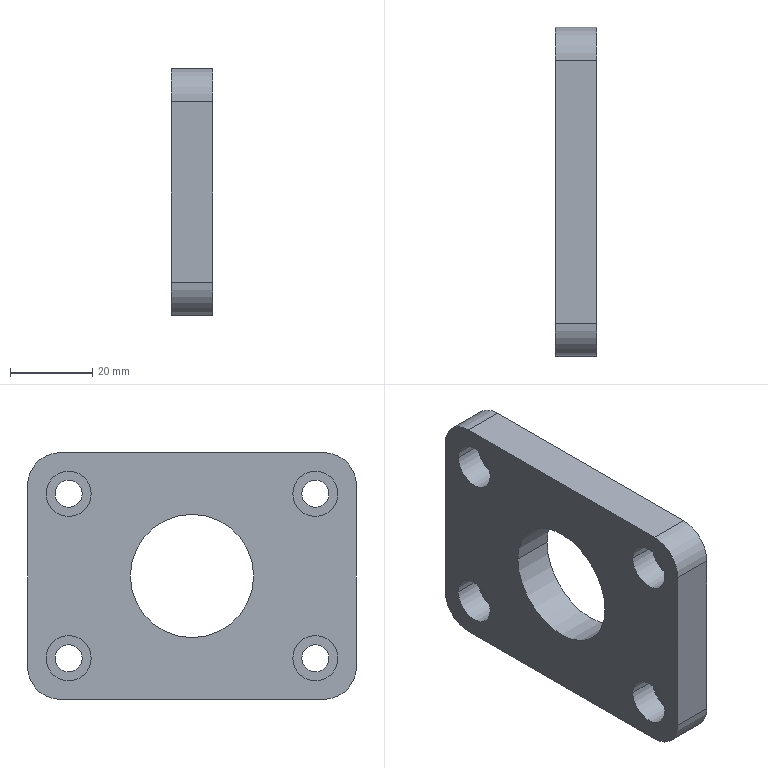Component | SolidWorks | GuideWheelAssembly-2_GuideWheelBracket-1_GuideWheelBracketPlate-1 | 1 solid | 32 faces | box 10 x 80 x 60 mm | volume 37359 mm3 | cylinder 22 | plane 10 | commonest cylinder face diameters 11 x8 6.6 x8 16 x4 30 x2 | material Nylon 101
build123d program:
from build123d import *

# Parameters (mm, degrees)
SKETCH1_W                                            = 80
SKETCH1_H                                            = 60
BOSS_EXTRUDE1_DEPTH                                  = 10
FILLET1_R                                            = 8
HOLE_SIZE_ACCORDING_TO_THE_TYPE_OF_HEXAG_D           = 6.6
HOLE_SIZE_ACCORDING_TO_THE_TYPE_OF_HEXAG_CBORE_D     = 11
HOLE_SIZE_ACCORDING_TO_THE_TYPE_OF_HEXAG_CBORE_DEPTH = 6.8
SKETCH4_R                                            = 15
CUT_EXTRUDE1_DEPTH                                   = 10


with BuildPart() as part:
    # Sketch1 → Boss-Extrude1 (new body)
    with BuildSketch(Plane.XY):
        Rectangle(SKETCH1_W, SKETCH1_H)
    extrude(amount=BOSS_EXTRUDE1_DEPTH)

    # Fillet1
    fillet1_edges = [part.edges().sort_by_distance(p)[0] for p in [
        (40, -30, 5),
        (-40, -30, 5),
        (-40, 30, 5),
        (40, 30, 5),
    ]]
    fillet(fillet1_edges, radius=FILLET1_R)

    # Hole Size according to the type of Hexag (through all)
    with Locations(Plane.XY.offset(10)):
        with Locations((-30, 20), (30, 20), (-30, -20), (30, -20)):
            CounterBoreHole(HOLE_SIZE_ACCORDING_TO_THE_TYPE_OF_HEXAG_D / 2, HOLE_SIZE_ACCORDING_TO_THE_TYPE_OF_HEXAG_CBORE_D / 2, HOLE_SIZE_ACCORDING_TO_THE_TYPE_OF_HEXAG_CBORE_DEPTH)

    # Sketch4 → Cut-Extrude1 (cut)
    with BuildSketch(Plane.XY.offset(10)):
        Circle(SKETCH4_R)
    extrude(amount=-CUT_EXTRUDE1_DEPTH, mode=Mode.SUBTRACT)


solid = part.part

# Placed as in the assembly
solid = solid.moved(Location((-510, 0, 305), (90, -90, 0)))
STEP:
#1=COLOUR_RGB('',0.7922,0.8196,0.9333);
#2=FILL_AREA_STYLE_COLOUR('',#1);
#3=FILL_AREA_STYLE('',(#2));
#4=SURFACE_STYLE_FILL_AREA(#3);
#5=SURFACE_SIDE_STYLE('',(#4));
#6=SURFACE_STYLE_USAGE(.BOTH.,#5);
#7=PRESENTATION_STYLE_ASSIGNMENT((#6));
#8=CARTESIAN_POINT('',(-20.079,0.5906,12.008));
#9=VERTEX_POINT('',#8);
#10=CARTESIAN_POINT('',(-20.079,-0.5906,12.008));
#11=VERTEX_POINT('',#10);
#12=CARTESIAN_POINT('',(-20.079,-0.,12.008));
#13=DIRECTION('',(-1.,0.,-0.));
#14=DIRECTION('',(0.,-1.,0.));
#15=AXIS2_PLACEMENT_3D('',#12,#13,#14);
#16=CIRCLE('',#15,0.5906);
#17=EDGE_CURVE('',#9,#11,#16,.T.);
#18=ORIENTED_EDGE('',*,*,#17,.F.);
#19=CARTESIAN_POINT('',(-20.472,0.5906,12.008));
#20=VERTEX_POINT('',#19);
#21=CARTESIAN_POINT('',(-20.079,0.5906,12.008));
#22=DIRECTION('',(-1.,0.,-0.));
#23=VECTOR('',#22,39.37);
#24=LINE('',#21,#23);
#25=EDGE_CURVE('',#9,#20,#24,.T.);
#26=ORIENTED_EDGE('',*,*,#25,.T.);
#27=CARTESIAN_POINT('',(-20.472,-0.5906,12.008));
#28=VERTEX_POINT('',#27);
#29=CARTESIAN_POINT('',(-20.472,-0.,12.008));
#30=DIRECTION('',(-1.,0.,-0.));
#31=DIRECTION('',(0.,-1.,0.));
#32=AXIS2_PLACEMENT_3D('',#29,#30,#31);
#33=CIRCLE('',#32,0.5906);
#34=EDGE_CURVE('',#20,#28,#33,.T.);
#35=ORIENTED_EDGE('',*,*,#34,.T.);
#36=CARTESIAN_POINT('',(-20.079,-0.5906,12.008));
#37=DIRECTION('',(-1.,0.,-0.));
#38=VECTOR('',#37,39.37);
#39=LINE('',#36,#38);
#40=EDGE_CURVE('',#11,#28,#39,.T.);
#41=ORIENTED_EDGE('',*,*,#40,.F.);
#42=EDGE_LOOP('',(#18,#26,#35,#41));
#43=FACE_OUTER_BOUND('',#42,.T.);
#44=CARTESIAN_POINT('',(-20.079,-0.,12.008));
#45=DIRECTION('',(-1.,0.,-0.));
#46=DIRECTION('',(0.,-1.,0.));
#47=AXIS2_PLACEMENT_3D('',#44,#45,#46);
#48=CYLINDRICAL_SURFACE('',#47,0.5906);
#49=ADVANCED_FACE('',(#43),#48,.F.);
#50=CARTESIAN_POINT('',(-20.205,1.398,12.795));
#51=VERTEX_POINT('',#50);
#52=CARTESIAN_POINT('',(-20.205,0.9646,12.795));
#53=VERTEX_POINT('',#52);
#54=CARTESIAN_POINT('',(-20.205,1.181,12.795));
#55=DIRECTION('',(-1.,0.,-0.));
#56=DIRECTION('',(0.,-1.,0.));
#57=AXIS2_PLACEMENT_3D('',#54,#55,#56);
#58=CIRCLE('',#57,0.2165);
#59=EDGE_CURVE('',#51,#53,#58,.T.);
#60=ORIENTED_EDGE('',*,*,#59,.F.);
#61=CARTESIAN_POINT('',(-20.472,1.398,12.795));
#62=VERTEX_POINT('',#61);
#63=CARTESIAN_POINT('',(-20.472,1.398,12.795));
#64=DIRECTION('',(-1.,0.,-0.));
#65=VECTOR('',#64,39.37);
#66=LINE('',#63,#65);
#67=EDGE_CURVE('',#51,#62,#66,.T.);
#68=ORIENTED_EDGE('',*,*,#67,.T.);
#69=CARTESIAN_POINT('',(-20.472,0.9646,12.795));
#70=VERTEX_POINT('',#69);
#71=CARTESIAN_POINT('',(-20.472,1.181,12.795));
#72=DIRECTION('',(-1.,0.,-0.));
#73=DIRECTION('',(0.,-1.,0.));
#74=AXIS2_PLACEMENT_3D('',#71,#72,#73);
#75=CIRCLE('',#74,0.2165);
#76=EDGE_CURVE('',#62,#70,#75,.T.);
#77=ORIENTED_EDGE('',*,*,#76,.T.);
#78=CARTESIAN_POINT('',(-20.472,0.9646,12.795));
#79=DIRECTION('',(-1.,0.,-0.));
#80=VECTOR('',#79,39.37);
#81=LINE('',#78,#80);
#82=EDGE_CURVE('',#53,#70,#81,.T.);
#83=ORIENTED_EDGE('',*,*,#82,.F.);
#84=EDGE_LOOP('',(#60,#68,#77,#83));
#85=FACE_OUTER_BOUND('',#84,.T.);
#86=CARTESIAN_POINT('',(-20.472,1.181,12.795));
#87=DIRECTION('',(-1.,0.,-0.));
#88=DIRECTION('',(0.,-1.,0.));
#89=AXIS2_PLACEMENT_3D('',#86,#87,#88);
#90=CYLINDRICAL_SURFACE('',#89,0.2165);
#91=ADVANCED_FACE('',(#85),#90,.F.);
#92=CARTESIAN_POINT('',(-20.079,1.311,12.795));
#93=VERTEX_POINT('',#92);
#94=CARTESIAN_POINT('',(-20.079,1.051,12.795));
#95=VERTEX_POINT('',#94);
#96=CARTESIAN_POINT('',(-20.079,1.181,12.795));
#97=DIRECTION('',(-1.,0.,-0.));
#98=DIRECTION('',(0.,-1.,0.));
#99=AXIS2_PLACEMENT_3D('',#96,#97,#98);
#100=CIRCLE('',#99,0.1299);
#101=EDGE_CURVE('',#93,#95,#100,.T.);
#102=ORIENTED_EDGE('',*,*,#101,.F.);
#103=CARTESIAN_POINT('',(-20.205,1.311,12.795));
#104=VERTEX_POINT('',#103);
#105=CARTESIAN_POINT('',(-20.472,1.311,12.795));
#106=DIRECTION('',(-1.,0.,-0.));
#107=VECTOR('',#106,39.37);
#108=LINE('',#105,#107);
#109=EDGE_CURVE('',#93,#104,#108,.T.);
#110=ORIENTED_EDGE('',*,*,#109,.T.);
#111=CARTESIAN_POINT('',(-20.205,1.051,12.795));
#112=VERTEX_POINT('',#111);
#113=CARTESIAN_POINT('',(-20.205,1.181,12.795));
#114=DIRECTION('',(-1.,0.,-0.));
#115=DIRECTION('',(0.,-1.,0.));
#116=AXIS2_PLACEMENT_3D('',#113,#114,#115);
#117=CIRCLE('',#116,0.1299);
#118=EDGE_CURVE('',#104,#112,#117,.T.);
#119=ORIENTED_EDGE('',*,*,#118,.T.);
#120=CARTESIAN_POINT('',(-20.472,1.051,12.795));
#121=DIRECTION('',(-1.,0.,-0.));
#122=VECTOR('',#121,39.37);
#123=LINE('',#120,#122);
#124=EDGE_CURVE('',#95,#112,#123,.T.);
#125=ORIENTED_EDGE('',*,*,#124,.F.);
#126=EDGE_LOOP('',(#102,#110,#119,#125));
#127=FACE_OUTER_BOUND('',#126,.T.);
#128=CARTESIAN_POINT('',(-20.472,1.181,12.795));
#129=DIRECTION('',(-1.,0.,-0.));
#130=DIRECTION('',(0.,-1.,0.));
#131=AXIS2_PLACEMENT_3D('',#128,#129,#130);
#132=CYLINDRICAL_SURFACE('',#131,0.1299);
#133=ADVANCED_FACE('',(#127),#132,.F.);
#134=CARTESIAN_POINT('',(-20.205,-0.9646,12.795));
#135=VERTEX_POINT('',#134);
#136=CARTESIAN_POINT('',(-20.205,-1.398,12.795));
#137=VERTEX_POINT('',#136);
#138=CARTESIAN_POINT('',(-20.205,-1.181,12.795));
#139=DIRECTION('',(-1.,0.,-0.));
#140=DIRECTION('',(0.,-1.,0.));
#141=AXIS2_PLACEMENT_3D('',#138,#139,#140);
#142=CIRCLE('',#141,0.2165);
#143=EDGE_CURVE('',#135,#137,#142,.T.);
#144=ORIENTED_EDGE('',*,*,#143,.F.);
#145=CARTESIAN_POINT('',(-20.472,-0.9646,12.795));
#146=VERTEX_POINT('',#145);
#147=CARTESIAN_POINT('',(-20.472,-0.9646,12.795));
#148=DIRECTION('',(-1.,0.,-0.));
#149=VECTOR('',#148,39.37);
#150=LINE('',#147,#149);
#151=EDGE_CURVE('',#135,#146,#150,.T.);
#152=ORIENTED_EDGE('',*,*,#151,.T.);
#153=CARTESIAN_POINT('',(-20.472,-1.398,12.795));
#154=VERTEX_POINT('',#153);
#155=CARTESIAN_POINT('',(-20.472,-1.181,12.795));
#156=DIRECTION('',(-1.,0.,-0.));
#157=DIRECTION('',(0.,-1.,0.));
#158=AXIS2_PLACEMENT_3D('',#155,#156,#157);
#159=CIRCLE('',#158,0.2165);
#160=EDGE_CURVE('',#146,#154,#159,.T.);
#161=ORIENTED_EDGE('',*,*,#160,.T.);
#162=CARTESIAN_POINT('',(-20.472,-1.398,12.795));
#163=DIRECTION('',(-1.,0.,-0.));
#164=VECTOR('',#163,39.37);
#165=LINE('',#162,#164);
#166=EDGE_CURVE('',#137,#154,#165,.T.);
#167=ORIENTED_EDGE('',*,*,#166,.F.);
#168=EDGE_LOOP('',(#144,#152,#161,#167));
#169=FACE_OUTER_BOUND('',#168,.T.);
#170=CARTESIAN_POINT('',(-20.472,-1.181,12.795));
#171=DIRECTION('',(-1.,0.,-0.));
#172=DIRECTION('',(0.,-1.,0.));
#173=AXIS2_PLACEMENT_3D('',#170,#171,#172);
#174=CYLINDRICAL_SURFACE('',#173,0.2165);
#175=ADVANCED_FACE('',(#169),#174,.F.);
#176=CARTESIAN_POINT('',(-20.079,-1.051,12.795));
#177=VERTEX_POINT('',#176);
#178=CARTESIAN_POINT('',(-20.079,-1.311,12.795));
#179=VERTEX_POINT('',#178);
#180=CARTESIAN_POINT('',(-20.079,-1.181,12.795));
#181=DIRECTION('',(-1.,0.,-0.));
#182=DIRECTION('',(0.,-1.,0.));
#183=AXIS2_PLACEMENT_3D('',#180,#181,#182);
#184=CIRCLE('',#183,0.1299);
#185=EDGE_CURVE('',#177,#179,#184,.T.);
#186=ORIENTED_EDGE('',*,*,#185,.F.);
#187=CARTESIAN_POINT('',(-20.205,-1.051,12.795));
#188=VERTEX_POINT('',#187);
#189=CARTESIAN_POINT('',(-20.472,-1.051,12.795));
#190=DIRECTION('',(-1.,0.,-0.));
#191=VECTOR('',#190,39.37);
#192=LINE('',#189,#191);
#193=EDGE_CURVE('',#177,#188,#192,.T.);
#194=ORIENTED_EDGE('',*,*,#193,.T.);
#195=CARTESIAN_POINT('',(-20.205,-1.311,12.795));
#196=VERTEX_POINT('',#195);
#197=CARTESIAN_POINT('',(-20.205,-1.181,12.795));
#198=DIRECTION('',(-1.,0.,-0.));
#199=DIRECTION('',(0.,-1.,0.));
#200=AXIS2_PLACEMENT_3D('',#197,#198,#199);
#201=CIRCLE('',#200,0.1299);
#202=EDGE_CURVE('',#188,#196,#201,.T.);
#203=ORIENTED_EDGE('',*,*,#202,.T.);
#204=CARTESIAN_POINT('',(-20.472,-1.311,12.795));
#205=DIRECTION('',(-1.,0.,-0.));
#206=VECTOR('',#205,39.37);
#207=LINE('',#204,#206);
#208=EDGE_CURVE('',#179,#196,#207,.T.);
#209=ORIENTED_EDGE('',*,*,#208,.F.);
#210=EDGE_LOOP('',(#186,#194,#203,#209));
#211=FACE_OUTER_BOUND('',#210,.T.);
#212=CARTESIAN_POINT('',(-20.472,-1.181,12.795));
#213=DIRECTION('',(-1.,0.,-0.));
#214=DIRECTION('',(0.,-1.,0.));
#215=AXIS2_PLACEMENT_3D('',#212,#213,#214);
#216=CYLINDRICAL_SURFACE('',#215,0.1299);
#217=ADVANCED_FACE('',(#211),#216,.F.);
#218=CARTESIAN_POINT('',(-20.205,1.398,11.22));
#219=VERTEX_POINT('',#218);
#220=CARTESIAN_POINT('',(-20.205,0.9646,11.22));
#221=VERTEX_POINT('',#220);
#222=CARTESIAN_POINT('',(-20.205,1.181,11.22));
#223=DIRECTION('',(-1.,0.,-0.));
#224=DIRECTION('',(0.,-1.,0.));
#225=AXIS2_PLACEMENT_3D('',#222,#223,#224);
#226=CIRCLE('',#225,0.2165);
#227=EDGE_CURVE('',#219,#221,#226,.T.);
#228=ORIENTED_EDGE('',*,*,#227,.F.);
#229=CARTESIAN_POINT('',(-20.472,1.398,11.22));
#230=VERTEX_POINT('',#229);
#231=CARTESIAN_POINT('',(-20.472,1.398,11.22));
#232=DIRECTION('',(-1.,0.,-0.));
#233=VECTOR('',#232,39.37);
#234=LINE('',#231,#233);
#235=EDGE_CURVE('',#219,#230,#234,.T.);
#236=ORIENTED_EDGE('',*,*,#235,.T.);
#237=CARTESIAN_POINT('',(-20.472,0.9646,11.22));
#238=VERTEX_POINT('',#237);
#239=CARTESIAN_POINT('',(-20.472,1.181,11.22));
#240=DIRECTION('',(-1.,0.,-0.));
#241=DIRECTION('',(0.,-1.,0.));
#242=AXIS2_PLACEMENT_3D('',#239,#240,#241);
#243=CIRCLE('',#242,0.2165);
#244=EDGE_CURVE('',#230,#238,#243,.T.);
#245=ORIENTED_EDGE('',*,*,#244,.T.);
#246=CARTESIAN_POINT('',(-20.472,0.9646,11.22));
#247=DIRECTION('',(-1.,0.,-0.));
#248=VECTOR('',#247,39.37);
#249=LINE('',#246,#248);
#250=EDGE_CURVE('',#221,#238,#249,.T.);
#251=ORIENTED_EDGE('',*,*,#250,.F.);
#252=EDGE_LOOP('',(#228,#236,#245,#251));
#253=FACE_OUTER_BOUND('',#252,.T.);
#254=CARTESIAN_POINT('',(-20.472,1.181,11.22));
#255=DIRECTION('',(-1.,0.,-0.));
#256=DIRECTION('',(0.,-1.,0.));
#257=AXIS2_PLACEMENT_3D('',#254,#255,#256);
#258=CYLINDRICAL_SURFACE('',#257,0.2165);
#259=ADVANCED_FACE('',(#253),#258,.F.);
#260=CARTESIAN_POINT('',(-20.079,1.311,11.22));
#261=VERTEX_POINT('',#260);
#262=CARTESIAN_POINT('',(-20.079,1.051,11.22));
#263=VERTEX_POINT('',#262);
#264=CARTESIAN_POINT('',(-20.079,1.181,11.22));
#265=DIRECTION('',(-1.,0.,-0.));
#266=DIRECTION('',(0.,-1.,0.));
#267=AXIS2_PLACEMENT_3D('',#264,#265,#266);
#268=CIRCLE('',#267,0.1299);
#269=EDGE_CURVE('',#261,#263,#268,.T.);
#270=ORIENTED_EDGE('',*,*,#269,.F.);
#271=CARTESIAN_POINT('',(-20.205,1.311,11.22));
#272=VERTEX_POINT('',#271);
#273=CARTESIAN_POINT('',(-20.472,1.311,11.22));
#274=DIRECTION('',(-1.,0.,-0.));
#275=VECTOR('',#274,39.37);
#276=LINE('',#273,#275);
#277=EDGE_CURVE('',#261,#272,#276,.T.);
#278=ORIENTED_EDGE('',*,*,#277,.T.);
#279=CARTESIAN_POINT('',(-20.205,1.051,11.22));
#280=VERTEX_POINT('',#279);
#281=CARTESIAN_POINT('',(-20.205,1.181,11.22));
#282=DIRECTION('',(-1.,0.,-0.));
#283=DIRECTION('',(0.,-1.,0.));
#284=AXIS2_PLACEMENT_3D('',#281,#282,#283);
#285=CIRCLE('',#284,0.1299);
#286=EDGE_CURVE('',#272,#280,#285,.T.);
#287=ORIENTED_EDGE('',*,*,#286,.T.);
#288=CARTESIAN_POINT('',(-20.472,1.051,11.22));
#289=DIRECTION('',(-1.,0.,-0.));
#290=VECTOR('',#289,39.37);
#291=LINE('',#288,#290);
#292=EDGE_CURVE('',#263,#280,#291,.T.);
#293=ORIENTED_EDGE('',*,*,#292,.F.);
#294=EDGE_LOOP('',(#270,#278,#287,#293));
#295=FACE_OUTER_BOUND('',#294,.T.);
#296=CARTESIAN_POINT('',(-20.472,1.181,11.22));
#297=DIRECTION('',(-1.,0.,-0.));
#298=DIRECTION('',(0.,-1.,0.));
#299=AXIS2_PLACEMENT_3D('',#296,#297,#298);
#300=CYLINDRICAL_SURFACE('',#299,0.1299);
#301=ADVANCED_FACE('',(#295),#300,.F.);
#302=CARTESIAN_POINT('',(-20.205,-0.9646,11.22));
#303=VERTEX_POINT('',#302);
#304=CARTESIAN_POINT('',(-20.205,-1.398,11.22));
#305=VERTEX_POINT('',#304);
#306=CARTESIAN_POINT('',(-20.205,-1.181,11.22));
#307=DIRECTION('',(-1.,0.,-0.));
#308=DIRECTION('',(0.,-1.,0.));
#309=AXIS2_PLACEMENT_3D('',#306,#307,#308);
#310=CIRCLE('',#309,0.2165);
#311=EDGE_CURVE('',#303,#305,#310,.T.);
#312=ORIENTED_EDGE('',*,*,#311,.F.);
#313=CARTESIAN_POINT('',(-20.472,-0.9646,11.22));
#314=VERTEX_POINT('',#313);
#315=CARTESIAN_POINT('',(-20.472,-0.9646,11.22));
#316=DIRECTION('',(-1.,0.,-0.));
#317=VECTOR('',#316,39.37);
#318=LINE('',#315,#317);
#319=EDGE_CURVE('',#303,#314,#318,.T.);
#320=ORIENTED_EDGE('',*,*,#319,.T.);
#321=CARTESIAN_POINT('',(-20.472,-1.398,11.22));
#322=VERTEX_POINT('',#321);
#323=CARTESIAN_POINT('',(-20.472,-1.181,11.22));
#324=DIRECTION('',(-1.,0.,-0.));
#325=DIRECTION('',(0.,-1.,0.));
#326=AXIS2_PLACEMENT_3D('',#323,#324,#325);
#327=CIRCLE('',#326,0.2165);
#328=EDGE_CURVE('',#314,#322,#327,.T.);
#329=ORIENTED_EDGE('',*,*,#328,.T.);
#330=CARTESIAN_POINT('',(-20.472,-1.398,11.22));
#331=DIRECTION('',(-1.,0.,-0.));
#332=VECTOR('',#331,39.37);
#333=LINE('',#330,#332);
#334=EDGE_CURVE('',#305,#322,#333,.T.);
#335=ORIENTED_EDGE('',*,*,#334,.F.);
#336=EDGE_LOOP('',(#312,#320,#329,#335));
#337=FACE_OUTER_BOUND('',#336,.T.);
#338=CARTESIAN_POINT('',(-20.472,-1.181,11.22));
#339=DIRECTION('',(-1.,0.,-0.));
#340=DIRECTION('',(0.,-1.,0.));
#341=AXIS2_PLACEMENT_3D('',#338,#339,#340);
#342=CYLINDRICAL_SURFACE('',#341,0.2165);
#343=ADVANCED_FACE('',(#337),#342,.F.);
#344=CARTESIAN_POINT('',(-20.079,-1.051,11.22));
#345=VERTEX_POINT('',#344);
#346=CARTESIAN_POINT('',(-20.079,-1.311,11.22));
#347=VERTEX_POINT('',#346);
#348=CARTESIAN_POINT('',(-20.079,-1.181,11.22));
#349=DIRECTION('',(-1.,0.,-0.));
#350=DIRECTION('',(0.,-1.,0.));
#351=AXIS2_PLACEMENT_3D('',#348,#349,#350);
#352=CIRCLE('',#351,0.1299);
#353=EDGE_CURVE('',#345,#347,#352,.T.);
#354=ORIENTED_EDGE('',*,*,#353,.F.);
#355=CARTESIAN_POINT('',(-20.205,-1.051,11.22));
#356=VERTEX_POINT('',#355);
#357=CARTESIAN_POINT('',(-20.472,-1.051,11.22));
#358=DIRECTION('',(-1.,0.,-0.));
#359=VECTOR('',#358,39.37);
#360=LINE('',#357,#359);
#361=EDGE_CURVE('',#345,#356,#360,.T.);
#362=ORIENTED_EDGE('',*,*,#361,.T.);
#363=CARTESIAN_POINT('',(-20.205,-1.311,11.22));
#364=VERTEX_POINT('',#363);
#365=CARTESIAN_POINT('',(-20.205,-1.181,11.22));
#366=DIRECTION('',(-1.,0.,-0.));
#367=DIRECTION('',(0.,-1.,0.));
#368=AXIS2_PLACEMENT_3D('',#365,#366,#367);
#369=CIRCLE('',#368,0.1299);
#370=EDGE_CURVE('',#356,#364,#369,.T.);
#371=ORIENTED_EDGE('',*,*,#370,.T.);
#372=CARTESIAN_POINT('',(-20.472,-1.311,11.22));
#373=DIRECTION('',(-1.,0.,-0.));
#374=VECTOR('',#373,39.37);
#375=LINE('',#372,#374);
#376=EDGE_CURVE('',#347,#364,#375,.T.);
#377=ORIENTED_EDGE('',*,*,#376,.F.);
#378=EDGE_LOOP('',(#354,#362,#371,#377));
#379=FACE_OUTER_BOUND('',#378,.T.);
#380=CARTESIAN_POINT('',(-20.472,-1.181,11.22));
#381=DIRECTION('',(-1.,0.,-0.));
#382=DIRECTION('',(0.,-1.,0.));
#383=AXIS2_PLACEMENT_3D('',#380,#381,#382);
#384=CYLINDRICAL_SURFACE('',#383,0.1299);
#385=ADVANCED_FACE('',(#379),#384,.F.);
#386=CARTESIAN_POINT('',(-20.472,-1.575,11.142));
#387=VERTEX_POINT('',#386);
#388=CARTESIAN_POINT('',(-20.472,-1.575,12.874));
#389=VERTEX_POINT('',#388);
#390=CARTESIAN_POINT('',(-20.472,-1.575,13.189));
#391=DIRECTION('',(-0.,-0.,1.));
#392=VECTOR('',#391,39.37);
#393=LINE('',#390,#392);
#394=EDGE_CURVE('',#387,#389,#393,.T.);
#395=ORIENTED_EDGE('',*,*,#394,.F.);
#396=CARTESIAN_POINT('',(-20.079,-1.575,11.142));
#397=VERTEX_POINT('',#396);
#398=CARTESIAN_POINT('',(-20.472,-1.575,11.142));
#399=DIRECTION('',(1.,-0.,0.));
#400=VECTOR('',#399,39.37);
#401=LINE('',#398,#400);
#402=EDGE_CURVE('',#387,#397,#401,.T.);
#403=ORIENTED_EDGE('',*,*,#402,.T.);
#404=CARTESIAN_POINT('',(-20.079,-1.575,12.874));
#405=VERTEX_POINT('',#404);
#406=CARTESIAN_POINT('',(-20.079,-1.575,13.189));
#407=DIRECTION('',(-0.,-0.,1.));
#408=VECTOR('',#407,39.37);
#409=LINE('',#406,#408);
#410=EDGE_CURVE('',#397,#405,#409,.T.);
#411=ORIENTED_EDGE('',*,*,#410,.T.);
#412=CARTESIAN_POINT('',(-20.472,-1.575,12.874));
#413=DIRECTION('',(-1.,0.,-0.));
#414=VECTOR('',#413,39.37);
#415=LINE('',#412,#414);
#416=EDGE_CURVE('',#405,#389,#415,.T.);
#417=ORIENTED_EDGE('',*,*,#416,.T.);
#418=EDGE_LOOP('',(#395,#403,#411,#417));
#419=FACE_OUTER_BOUND('',#418,.T.);
#420=CARTESIAN_POINT('',(-20.472,-1.575,13.189));
#421=DIRECTION('',(-0.,1.,0.));
#422=DIRECTION('',(0.,0.,-1.));
#423=AXIS2_PLACEMENT_3D('',#420,#421,#422);
#424=PLANE('',#423);
#425=ADVANCED_FACE('',(#419),#424,.F.);
#426=CARTESIAN_POINT('',(-20.079,-1.26,13.189));
#427=VERTEX_POINT('',#426);
#428=CARTESIAN_POINT('',(-20.079,1.26,13.189));
#429=VERTEX_POINT('',#428);
#430=CARTESIAN_POINT('',(-20.079,1.575,13.189));
#431=DIRECTION('',(-0.,1.,0.));
#432=VECTOR('',#431,39.37);
#433=LINE('',#430,#432);
#434=EDGE_CURVE('',#427,#429,#433,.T.);
#435=ORIENTED_EDGE('',*,*,#434,.T.);
#436=CARTESIAN_POINT('',(-20.472,1.26,13.189));
#437=VERTEX_POINT('',#436);
#438=CARTESIAN_POINT('',(-20.472,1.26,13.189));
#439=DIRECTION('',(-1.,0.,-0.));
#440=VECTOR('',#439,39.37);
#441=LINE('',#438,#440);
#442=EDGE_CURVE('',#429,#437,#441,.T.);
#443=ORIENTED_EDGE('',*,*,#442,.T.);
#444=CARTESIAN_POINT('',(-20.472,-1.26,13.189));
#445=VERTEX_POINT('',#444);
#446=CARTESIAN_POINT('',(-20.472,1.575,13.189));
#447=DIRECTION('',(-0.,1.,0.));
#448=VECTOR('',#447,39.37);
#449=LINE('',#446,#448);
#450=EDGE_CURVE('',#445,#437,#449,.T.);
#451=ORIENTED_EDGE('',*,*,#450,.F.);
#452=CARTESIAN_POINT('',(-20.472,-1.26,13.189));
#453=DIRECTION('',(1.,-0.,0.));
#454=VECTOR('',#453,39.37);
#455=LINE('',#452,#454);
#456=EDGE_CURVE('',#445,#427,#455,.T.);
#457=ORIENTED_EDGE('',*,*,#456,.T.);
#458=EDGE_LOOP('',(#435,#443,#451,#457));
#459=FACE_OUTER_BOUND('',#458,.T.);
#460=CARTESIAN_POINT('',(-20.472,1.575,13.189));
#461=DIRECTION('',(0.,0.,-1.));
#462=DIRECTION('',(1.,-0.,0.));
#463=AXIS2_PLACEMENT_3D('',#460,#461,#462);
#464=PLANE('',#463);
#465=ADVANCED_FACE('',(#459),#464,.F.);
#466=CARTESIAN_POINT('',(-20.079,1.575,12.874));
#467=VERTEX_POINT('',#466);
#468=CARTESIAN_POINT('',(-20.079,1.575,11.142));
#469=VERTEX_POINT('',#468);
#470=CARTESIAN_POINT('',(-20.079,1.575,13.189));
#471=DIRECTION('',(0.,0.,-1.));
#472=VECTOR('',#471,39.37);
#473=LINE('',#470,#472);
#474=EDGE_CURVE('',#467,#469,#473,.T.);
#475=ORIENTED_EDGE('',*,*,#474,.T.);
#476=CARTESIAN_POINT('',(-20.472,1.575,11.142));
#477=VERTEX_POINT('',#476);
#478=CARTESIAN_POINT('',(-20.472,1.575,11.142));
#479=DIRECTION('',(-1.,0.,-0.));
#480=VECTOR('',#479,39.37);
#481=LINE('',#478,#480);
#482=EDGE_CURVE('',#469,#477,#481,.T.);
#483=ORIENTED_EDGE('',*,*,#482,.T.);
#484=CARTESIAN_POINT('',(-20.472,1.575,12.874));
#485=VERTEX_POINT('',#484);
#486=CARTESIAN_POINT('',(-20.472,1.575,13.189));
#487=DIRECTION('',(0.,0.,-1.));
#488=VECTOR('',#487,39.37);
#489=LINE('',#486,#488);
#490=EDGE_CURVE('',#485,#477,#489,.T.);
#491=ORIENTED_EDGE('',*,*,#490,.F.);
#492=CARTESIAN_POINT('',(-20.472,1.575,12.874));
#493=DIRECTION('',(1.,-0.,0.));
#494=VECTOR('',#493,39.37);
#495=LINE('',#492,#494);
#496=EDGE_CURVE('',#485,#467,#495,.T.);
#497=ORIENTED_EDGE('',*,*,#496,.T.);
#498=EDGE_LOOP('',(#475,#483,#491,#497));
#499=FACE_OUTER_BOUND('',#498,.T.);
#500=CARTESIAN_POINT('',(-20.472,1.575,13.189));
#501=DIRECTION('',(0.,-1.,-0.));
#502=DIRECTION('',(-0.,-0.,1.));
#503=AXIS2_PLACEMENT_3D('',#500,#501,#502);
#504=PLANE('',#503);
#505=ADVANCED_FACE('',(#499),#504,.F.);
#506=CARTESIAN_POINT('',(-20.079,1.26,10.827));
#507=VERTEX_POINT('',#506);
#508=CARTESIAN_POINT('',(-20.079,-1.26,10.827));
#509=VERTEX_POINT('',#508);
#510=CARTESIAN_POINT('',(-20.079,1.575,10.827));
#511=DIRECTION('',(0.,-1.,-0.));
#512=VECTOR('',#511,39.37);
#513=LINE('',#510,#512);
#514=EDGE_CURVE('',#507,#509,#513,.T.);
#515=ORIENTED_EDGE('',*,*,#514,.T.);
#516=CARTESIAN_POINT('',(-20.472,-1.26,10.827));
#517=VERTEX_POINT('',#516);
#518=CARTESIAN_POINT('',(-20.472,-1.26,10.827));
#519=DIRECTION('',(-1.,0.,-0.));
#520=VECTOR('',#519,39.37);
#521=LINE('',#518,#520);
#522=EDGE_CURVE('',#509,#517,#521,.T.);
#523=ORIENTED_EDGE('',*,*,#522,.T.);
#524=CARTESIAN_POINT('',(-20.472,1.26,10.827));
#525=VERTEX_POINT('',#524);
#526=CARTESIAN_POINT('',(-20.472,1.575,10.827));
#527=DIRECTION('',(0.,-1.,-0.));
#528=VECTOR('',#527,39.37);
#529=LINE('',#526,#528);
#530=EDGE_CURVE('',#525,#517,#529,.T.);
#531=ORIENTED_EDGE('',*,*,#530,.F.);
#532=CARTESIAN_POINT('',(-20.472,1.26,10.827));
#533=DIRECTION('',(1.,-0.,0.));
#534=VECTOR('',#533,39.37);
#535=LINE('',#532,#534);
#536=EDGE_CURVE('',#525,#507,#535,.T.);
#537=ORIENTED_EDGE('',*,*,#536,.T.);
#538=EDGE_LOOP('',(#515,#523,#531,#537));
#539=FACE_OUTER_BOUND('',#538,.T.);
#540=CARTESIAN_POINT('',(-20.472,1.575,10.827));
#541=DIRECTION('',(-0.,-0.,1.));
#542=DIRECTION('',(-1.,0.,-0.));
#543=AXIS2_PLACEMENT_3D('',#540,#541,#542);
#544=PLANE('',#543);
#545=ADVANCED_FACE('',(#539),#544,.F.);
#546=CARTESIAN_POINT('',(-20.472,-0.,12.008));
#547=DIRECTION('',(-1.,0.,-0.));
#548=DIRECTION('',(0.,-1.,0.));
#549=AXIS2_PLACEMENT_3D('',#546,#547,#548);
#550=CIRCLE('',#549,0.5906);
#551=EDGE_CURVE('',#28,#20,#550,.T.);
#552=ORIENTED_EDGE('',*,*,#551,.F.);
#553=ORIENTED_EDGE('',*,*,#34,.F.);
#554=EDGE_LOOP('',(#552,#553));
#555=FACE_BOUND('',#554,.T.);
#556=CARTESIAN_POINT('',(-20.472,1.181,12.795));
#557=DIRECTION('',(-1.,0.,-0.));
#558=DIRECTION('',(0.,-1.,0.));
#559=AXIS2_PLACEMENT_3D('',#556,#557,#558);
#560=CIRCLE('',#559,0.2165);
#561=EDGE_CURVE('',#70,#62,#560,.T.);
#562=ORIENTED_EDGE('',*,*,#561,.F.);
#563=ORIENTED_EDGE('',*,*,#76,.F.);
#564=EDGE_LOOP('',(#562,#563));
#565=FACE_BOUND('',#564,.T.);
#566=CARTESIAN_POINT('',(-20.472,-1.181,12.795));
#567=DIRECTION('',(-1.,0.,-0.));
#568=DIRECTION('',(0.,-1.,0.));
#569=AXIS2_PLACEMENT_3D('',#566,#567,#568);
#570=CIRCLE('',#569,0.2165);
#571=EDGE_CURVE('',#154,#146,#570,.T.);
#572=ORIENTED_EDGE('',*,*,#571,.F.);
#573=ORIENTED_EDGE('',*,*,#160,.F.);
#574=EDGE_LOOP('',(#572,#573));
#575=FACE_BOUND('',#574,.T.);
#576=CARTESIAN_POINT('',(-20.472,1.181,11.22));
#577=DIRECTION('',(-1.,0.,-0.));
#578=DIRECTION('',(0.,-1.,0.));
#579=AXIS2_PLACEMENT_3D('',#576,#577,#578);
#580=CIRCLE('',#579,0.2165);
#581=EDGE_CURVE('',#238,#230,#580,.T.);
#582=ORIENTED_EDGE('',*,*,#581,.F.);
#583=ORIENTED_EDGE('',*,*,#244,.F.);
#584=EDGE_LOOP('',(#582,#583));
#585=FACE_BOUND('',#584,.T.);
#586=CARTESIAN_POINT('',(-20.472,-1.181,11.22));
#587=DIRECTION('',(-1.,0.,-0.));
#588=DIRECTION('',(0.,-1.,0.));
#589=AXIS2_PLACEMENT_3D('',#586,#587,#588);
#590=CIRCLE('',#589,0.2165);
#591=EDGE_CURVE('',#322,#314,#590,.T.);
#592=ORIENTED_EDGE('',*,*,#591,.F.);
#593=ORIENTED_EDGE('',*,*,#328,.F.);
#594=EDGE_LOOP('',(#592,#593));
#595=FACE_BOUND('',#594,.T.);
#596=ORIENTED_EDGE('',*,*,#530,.T.);
#597=CARTESIAN_POINT('',(-20.472,-1.26,11.142));
#598=DIRECTION('',(-1.,0.,-0.));
#599=DIRECTION('',(0.,-1.,0.));
#600=AXIS2_PLACEMENT_3D('',#597,#598,#599);
#601=CIRCLE('',#600,0.315);
#602=EDGE_CURVE('',#517,#387,#601,.T.);
#603=ORIENTED_EDGE('',*,*,#602,.T.);
#604=ORIENTED_EDGE('',*,*,#394,.T.);
#605=CARTESIAN_POINT('',(-20.472,-1.26,12.874));
#606=DIRECTION('',(-1.,0.,-0.));
#607=DIRECTION('',(0.,-1.,0.));
#608=AXIS2_PLACEMENT_3D('',#605,#606,#607);
#609=CIRCLE('',#608,0.315);
#610=EDGE_CURVE('',#389,#445,#609,.T.);
#611=ORIENTED_EDGE('',*,*,#610,.T.);
#612=ORIENTED_EDGE('',*,*,#450,.T.);
#613=CARTESIAN_POINT('',(-20.472,1.26,12.874));
#614=DIRECTION('',(-1.,0.,-0.));
#615=DIRECTION('',(0.,-1.,0.));
#616=AXIS2_PLACEMENT_3D('',#613,#614,#615);
#617=CIRCLE('',#616,0.315);
#618=EDGE_CURVE('',#437,#485,#617,.T.);
#619=ORIENTED_EDGE('',*,*,#618,.T.);
#620=ORIENTED_EDGE('',*,*,#490,.T.);
#621=CARTESIAN_POINT('',(-20.472,1.26,11.142));
#622=DIRECTION('',(-1.,0.,-0.));
#623=DIRECTION('',(0.,-1.,0.));
#624=AXIS2_PLACEMENT_3D('',#621,#622,#623);
#625=CIRCLE('',#624,0.315);
#626=EDGE_CURVE('',#477,#525,#625,.T.);
#627=ORIENTED_EDGE('',*,*,#626,.T.);
#628=EDGE_LOOP('',(#596,#603,#604,#611,#612,#619,#620,#627));
#629=FACE_OUTER_BOUND('',#628,.T.);
#630=CARTESIAN_POINT('',(-20.472,-0.,12.008));
#631=DIRECTION('',(-1.,-0.,-0.));
#632=DIRECTION('',(0.,-1.,-0.));
#633=AXIS2_PLACEMENT_3D('',#630,#631,#632);
#634=PLANE('',#633);
#635=ADVANCED_FACE('',(#555,#565,#575,#585,#595,#629),#634,.T.);
#636=CARTESIAN_POINT('',(-20.079,-0.,12.008));
#637=DIRECTION('',(-1.,0.,-0.));
#638=DIRECTION('',(0.,-1.,0.));
#639=AXIS2_PLACEMENT_3D('',#636,#637,#638);
#640=CIRCLE('',#639,0.5906);
#641=EDGE_CURVE('',#11,#9,#640,.T.);
#642=ORIENTED_EDGE('',*,*,#641,.T.);
#643=ORIENTED_EDGE('',*,*,#17,.T.);
#644=EDGE_LOOP('',(#642,#643));
#645=FACE_BOUND('',#644,.T.);
#646=CARTESIAN_POINT('',(-20.079,1.181,12.795));
#647=DIRECTION('',(-1.,0.,-0.));
#648=DIRECTION('',(0.,-1.,0.));
#649=AXIS2_PLACEMENT_3D('',#646,#647,#648);
#650=CIRCLE('',#649,0.1299);
#651=EDGE_CURVE('',#95,#93,#650,.T.);
#652=ORIENTED_EDGE('',*,*,#651,.T.);
#653=ORIENTED_EDGE('',*,*,#101,.T.);
#654=EDGE_LOOP('',(#652,#653));
#655=FACE_BOUND('',#654,.T.);
#656=CARTESIAN_POINT('',(-20.079,-1.181,12.795));
#657=DIRECTION('',(-1.,0.,-0.));
#658=DIRECTION('',(0.,-1.,0.));
#659=AXIS2_PLACEMENT_3D('',#656,#657,#658);
#660=CIRCLE('',#659,0.1299);
#661=EDGE_CURVE('',#179,#177,#660,.T.);
#662=ORIENTED_EDGE('',*,*,#661,.T.);
#663=ORIENTED_EDGE('',*,*,#185,.T.);
#664=EDGE_LOOP('',(#662,#663));
#665=FACE_BOUND('',#664,.T.);
#666=CARTESIAN_POINT('',(-20.079,1.181,11.22));
#667=DIRECTION('',(-1.,0.,-0.));
#668=DIRECTION('',(0.,-1.,0.));
#669=AXIS2_PLACEMENT_3D('',#666,#667,#668);
#670=CIRCLE('',#669,0.1299);
#671=EDGE_CURVE('',#263,#261,#670,.T.);
#672=ORIENTED_EDGE('',*,*,#671,.T.);
#673=ORIENTED_EDGE('',*,*,#269,.T.);
#674=EDGE_LOOP('',(#672,#673));
#675=FACE_BOUND('',#674,.T.);
#676=CARTESIAN_POINT('',(-20.079,-1.181,11.22));
#677=DIRECTION('',(-1.,0.,-0.));
#678=DIRECTION('',(0.,-1.,0.));
#679=AXIS2_PLACEMENT_3D('',#676,#677,#678);
#680=CIRCLE('',#679,0.1299);
#681=EDGE_CURVE('',#347,#345,#680,.T.);
#682=ORIENTED_EDGE('',*,*,#681,.T.);
#683=ORIENTED_EDGE('',*,*,#353,.T.);
#684=EDGE_LOOP('',(#682,#683));
#685=FACE_BOUND('',#684,.T.);
#686=ORIENTED_EDGE('',*,*,#410,.F.);
#687=CARTESIAN_POINT('',(-20.079,-1.26,11.142));
#688=DIRECTION('',(1.,-0.,0.));
#689=DIRECTION('',(0.,-1.,0.));
#690=AXIS2_PLACEMENT_3D('',#687,#688,#689);
#691=CIRCLE('',#690,0.315);
#692=EDGE_CURVE('',#397,#509,#691,.T.);
#693=ORIENTED_EDGE('',*,*,#692,.T.);
#694=ORIENTED_EDGE('',*,*,#514,.F.);
#695=CARTESIAN_POINT('',(-20.079,1.26,11.142));
#696=DIRECTION('',(1.,-0.,0.));
#697=DIRECTION('',(0.,-1.,0.));
#698=AXIS2_PLACEMENT_3D('',#695,#696,#697);
#699=CIRCLE('',#698,0.315);
#700=EDGE_CURVE('',#507,#469,#699,.T.);
#701=ORIENTED_EDGE('',*,*,#700,.T.);
#702=ORIENTED_EDGE('',*,*,#474,.F.);
#703=CARTESIAN_POINT('',(-20.079,1.26,12.874));
#704=DIRECTION('',(1.,-0.,0.));
#705=DIRECTION('',(0.,-1.,0.));
#706=AXIS2_PLACEMENT_3D('',#703,#704,#705);
#707=CIRCLE('',#706,0.315);
#708=EDGE_CURVE('',#467,#429,#707,.T.);
#709=ORIENTED_EDGE('',*,*,#708,.T.);
#710=ORIENTED_EDGE('',*,*,#434,.F.);
#711=CARTESIAN_POINT('',(-20.079,-1.26,12.874));
#712=DIRECTION('',(1.,-0.,0.));
#713=DIRECTION('',(0.,-1.,-0.));
#714=AXIS2_PLACEMENT_3D('',#711,#712,#713);
#715=CIRCLE('',#714,0.315);
#716=EDGE_CURVE('',#427,#405,#715,.T.);
#717=ORIENTED_EDGE('',*,*,#716,.T.);
#718=EDGE_LOOP('',(#686,#693,#694,#701,#702,#709,#710,#717));
#719=FACE_OUTER_BOUND('',#718,.T.);
#720=CARTESIAN_POINT('',(-20.079,-0.,12.008));
#721=DIRECTION('',(-1.,-0.,-0.));
#722=DIRECTION('',(0.,-1.,-0.));
#723=AXIS2_PLACEMENT_3D('',#720,#721,#722);
#724=PLANE('',#723);
#725=ADVANCED_FACE('',(#645,#655,#665,#675,#685,#719),#724,.F.);
#726=ORIENTED_EDGE('',*,*,#602,.F.);
#727=ORIENTED_EDGE('',*,*,#522,.F.);
#728=ORIENTED_EDGE('',*,*,#692,.F.);
#729=ORIENTED_EDGE('',*,*,#402,.F.);
#730=EDGE_LOOP('',(#726,#727,#728,#729));
#731=FACE_OUTER_BOUND('',#730,.T.);
#732=CARTESIAN_POINT('',(-20.472,-1.26,11.142));
#733=DIRECTION('',(1.,-0.,0.));
#734=DIRECTION('',(0.,1.,0.));
#735=AXIS2_PLACEMENT_3D('',#732,#733,#734);
#736=CYLINDRICAL_SURFACE('',#735,0.315);
#737=ADVANCED_FACE('',(#731),#736,.T.);
#738=ORIENTED_EDGE('',*,*,#626,.F.);
#739=ORIENTED_EDGE('',*,*,#482,.F.);
#740=ORIENTED_EDGE('',*,*,#700,.F.);
#741=ORIENTED_EDGE('',*,*,#536,.F.);
#742=EDGE_LOOP('',(#738,#739,#740,#741));
#743=FACE_OUTER_BOUND('',#742,.T.);
#744=CARTESIAN_POINT('',(-20.472,1.26,11.142));
#745=DIRECTION('',(1.,-0.,0.));
#746=DIRECTION('',(0.,1.,0.));
#747=AXIS2_PLACEMENT_3D('',#744,#745,#746);
#748=CYLINDRICAL_SURFACE('',#747,0.315);
#749=ADVANCED_FACE('',(#743),#748,.T.);
#750=ORIENTED_EDGE('',*,*,#618,.F.);
#751=ORIENTED_EDGE('',*,*,#442,.F.);
#752=ORIENTED_EDGE('',*,*,#708,.F.);
#753=ORIENTED_EDGE('',*,*,#496,.F.);
#754=EDGE_LOOP('',(#750,#751,#752,#753));
#755=FACE_OUTER_BOUND('',#754,.T.);
#756=CARTESIAN_POINT('',(-20.472,1.26,12.874));
#757=DIRECTION('',(1.,-0.,0.));
#758=DIRECTION('',(0.,1.,0.));
#759=AXIS2_PLACEMENT_3D('',#756,#757,#758);
#760=CYLINDRICAL_SURFACE('',#759,0.315);
#761=ADVANCED_FACE('',(#755),#760,.T.);
#762=ORIENTED_EDGE('',*,*,#610,.F.);
#763=ORIENTED_EDGE('',*,*,#416,.F.);
#764=ORIENTED_EDGE('',*,*,#716,.F.);
#765=ORIENTED_EDGE('',*,*,#456,.F.);
#766=EDGE_LOOP('',(#762,#763,#764,#765));
#767=FACE_OUTER_BOUND('',#766,.T.);
#768=CARTESIAN_POINT('',(-20.472,-1.26,12.874));
#769=DIRECTION('',(1.,-0.,0.));
#770=DIRECTION('',(0.,1.,0.));
#771=AXIS2_PLACEMENT_3D('',#768,#769,#770);
#772=CYLINDRICAL_SURFACE('',#771,0.315);
#773=ADVANCED_FACE('',(#767),#772,.T.);
#774=ORIENTED_EDGE('',*,*,#361,.F.);
#775=ORIENTED_EDGE('',*,*,#681,.F.);
#776=ORIENTED_EDGE('',*,*,#376,.T.);
#777=CARTESIAN_POINT('',(-20.205,-1.181,11.22));
#778=DIRECTION('',(-1.,0.,-0.));
#779=DIRECTION('',(0.,-1.,0.));
#780=AXIS2_PLACEMENT_3D('',#777,#778,#779);
#781=CIRCLE('',#780,0.1299);
#782=EDGE_CURVE('',#364,#356,#781,.T.);
#783=ORIENTED_EDGE('',*,*,#782,.T.);
#784=EDGE_LOOP('',(#774,#775,#776,#783));
#785=FACE_OUTER_BOUND('',#784,.T.);
#786=CARTESIAN_POINT('',(-20.472,-1.181,11.22));
#787=DIRECTION('',(-1.,0.,-0.));
#788=DIRECTION('',(0.,-1.,0.));
#789=AXIS2_PLACEMENT_3D('',#786,#787,#788);
#790=CYLINDRICAL_SURFACE('',#789,0.1299);
#791=ADVANCED_FACE('',(#785),#790,.F.);
#792=ORIENTED_EDGE('',*,*,#782,.F.);
#793=ORIENTED_EDGE('',*,*,#370,.F.);
#794=EDGE_LOOP('',(#792,#793));
#795=FACE_BOUND('',#794,.T.);
#796=CARTESIAN_POINT('',(-20.205,-1.181,11.22));
#797=DIRECTION('',(-1.,0.,-0.));
#798=DIRECTION('',(0.,-1.,0.));
#799=AXIS2_PLACEMENT_3D('',#796,#797,#798);
#800=CIRCLE('',#799,0.2165);
#801=EDGE_CURVE('',#305,#303,#800,.T.);
#802=ORIENTED_EDGE('',*,*,#801,.T.);
#803=ORIENTED_EDGE('',*,*,#311,.T.);
#804=EDGE_LOOP('',(#802,#803));
#805=FACE_OUTER_BOUND('',#804,.T.);
#806=CARTESIAN_POINT('',(-20.205,-1.311,11.22));
#807=DIRECTION('',(1.,0.,0.));
#808=DIRECTION('',(-0.,1.,0.));
#809=AXIS2_PLACEMENT_3D('',#806,#807,#808);
#810=PLANE('',#809);
#811=ADVANCED_FACE('',(#795,#805),#810,.F.);
#812=ORIENTED_EDGE('',*,*,#319,.F.);
#813=ORIENTED_EDGE('',*,*,#801,.F.);
#814=ORIENTED_EDGE('',*,*,#334,.T.);
#815=ORIENTED_EDGE('',*,*,#591,.T.);
#816=EDGE_LOOP('',(#812,#813,#814,#815));
#817=FACE_OUTER_BOUND('',#816,.T.);
#818=CARTESIAN_POINT('',(-20.472,-1.181,11.22));
#819=DIRECTION('',(-1.,0.,-0.));
#820=DIRECTION('',(0.,-1.,0.));
#821=AXIS2_PLACEMENT_3D('',#818,#819,#820);
#822=CYLINDRICAL_SURFACE('',#821,0.2165);
#823=ADVANCED_FACE('',(#817),#822,.F.);
#824=ORIENTED_EDGE('',*,*,#277,.F.);
#825=ORIENTED_EDGE('',*,*,#671,.F.);
#826=ORIENTED_EDGE('',*,*,#292,.T.);
#827=CARTESIAN_POINT('',(-20.205,1.181,11.22));
#828=DIRECTION('',(-1.,0.,-0.));
#829=DIRECTION('',(0.,-1.,0.));
#830=AXIS2_PLACEMENT_3D('',#827,#828,#829);
#831=CIRCLE('',#830,0.1299);
#832=EDGE_CURVE('',#280,#272,#831,.T.);
#833=ORIENTED_EDGE('',*,*,#832,.T.);
#834=EDGE_LOOP('',(#824,#825,#826,#833));
#835=FACE_OUTER_BOUND('',#834,.T.);
#836=CARTESIAN_POINT('',(-20.472,1.181,11.22));
#837=DIRECTION('',(-1.,0.,-0.));
#838=DIRECTION('',(0.,-1.,0.));
#839=AXIS2_PLACEMENT_3D('',#836,#837,#838);
#840=CYLINDRICAL_SURFACE('',#839,0.1299);
#841=ADVANCED_FACE('',(#835),#840,.F.);
#842=ORIENTED_EDGE('',*,*,#832,.F.);
#843=ORIENTED_EDGE('',*,*,#286,.F.);
#844=EDGE_LOOP('',(#842,#843));
#845=FACE_BOUND('',#844,.T.);
#846=CARTESIAN_POINT('',(-20.205,1.181,11.22));
#847=DIRECTION('',(-1.,0.,-0.));
#848=DIRECTION('',(0.,-1.,0.));
#849=AXIS2_PLACEMENT_3D('',#846,#847,#848);
#850=CIRCLE('',#849,0.2165);
#851=EDGE_CURVE('',#221,#219,#850,.T.);
#852=ORIENTED_EDGE('',*,*,#851,.T.);
#853=ORIENTED_EDGE('',*,*,#227,.T.);
#854=EDGE_LOOP('',(#852,#853));
#855=FACE_OUTER_BOUND('',#854,.T.);
#856=CARTESIAN_POINT('',(-20.205,1.051,11.22));
#857=DIRECTION('',(1.,0.,0.));
#858=DIRECTION('',(-0.,1.,0.));
#859=AXIS2_PLACEMENT_3D('',#856,#857,#858);
#860=PLANE('',#859);
#861=ADVANCED_FACE('',(#845,#855),#860,.F.);
#862=ORIENTED_EDGE('',*,*,#235,.F.);
#863=ORIENTED_EDGE('',*,*,#851,.F.);
#864=ORIENTED_EDGE('',*,*,#250,.T.);
#865=ORIENTED_EDGE('',*,*,#581,.T.);
#866=EDGE_LOOP('',(#862,#863,#864,#865));
#867=FACE_OUTER_BOUND('',#866,.T.);
#868=CARTESIAN_POINT('',(-20.472,1.181,11.22));
#869=DIRECTION('',(-1.,0.,-0.));
#870=DIRECTION('',(0.,-1.,0.));
#871=AXIS2_PLACEMENT_3D('',#868,#869,#870);
#872=CYLINDRICAL_SURFACE('',#871,0.2165);
#873=ADVANCED_FACE('',(#867),#872,.F.);
#874=ORIENTED_EDGE('',*,*,#193,.F.);
#875=ORIENTED_EDGE('',*,*,#661,.F.);
#876=ORIENTED_EDGE('',*,*,#208,.T.);
#877=CARTESIAN_POINT('',(-20.205,-1.181,12.795));
#878=DIRECTION('',(-1.,0.,-0.));
#879=DIRECTION('',(0.,-1.,0.));
#880=AXIS2_PLACEMENT_3D('',#877,#878,#879);
#881=CIRCLE('',#880,0.1299);
#882=EDGE_CURVE('',#196,#188,#881,.T.);
#883=ORIENTED_EDGE('',*,*,#882,.T.);
#884=EDGE_LOOP('',(#874,#875,#876,#883));
#885=FACE_OUTER_BOUND('',#884,.T.);
#886=CARTESIAN_POINT('',(-20.472,-1.181,12.795));
#887=DIRECTION('',(-1.,0.,-0.));
#888=DIRECTION('',(0.,-1.,0.));
#889=AXIS2_PLACEMENT_3D('',#886,#887,#888);
#890=CYLINDRICAL_SURFACE('',#889,0.1299);
#891=ADVANCED_FACE('',(#885),#890,.F.);
#892=ORIENTED_EDGE('',*,*,#882,.F.);
#893=ORIENTED_EDGE('',*,*,#202,.F.);
#894=EDGE_LOOP('',(#892,#893));
#895=FACE_BOUND('',#894,.T.);
#896=CARTESIAN_POINT('',(-20.205,-1.181,12.795));
#897=DIRECTION('',(-1.,0.,-0.));
#898=DIRECTION('',(0.,-1.,0.));
#899=AXIS2_PLACEMENT_3D('',#896,#897,#898);
#900=CIRCLE('',#899,0.2165);
#901=EDGE_CURVE('',#137,#135,#900,.T.);
#902=ORIENTED_EDGE('',*,*,#901,.T.);
#903=ORIENTED_EDGE('',*,*,#143,.T.);
#904=EDGE_LOOP('',(#902,#903));
#905=FACE_OUTER_BOUND('',#904,.T.);
#906=CARTESIAN_POINT('',(-20.205,-1.311,12.795));
#907=DIRECTION('',(1.,0.,0.));
#908=DIRECTION('',(-0.,1.,0.));
#909=AXIS2_PLACEMENT_3D('',#906,#907,#908);
#910=PLANE('',#909);
#911=ADVANCED_FACE('',(#895,#905),#910,.F.);
#912=ORIENTED_EDGE('',*,*,#151,.F.);
#913=ORIENTED_EDGE('',*,*,#901,.F.);
#914=ORIENTED_EDGE('',*,*,#166,.T.);
#915=ORIENTED_EDGE('',*,*,#571,.T.);
#916=EDGE_LOOP('',(#912,#913,#914,#915));
#917=FACE_OUTER_BOUND('',#916,.T.);
#918=CARTESIAN_POINT('',(-20.472,-1.181,12.795));
#919=DIRECTION('',(-1.,0.,-0.));
#920=DIRECTION('',(0.,-1.,0.));
#921=AXIS2_PLACEMENT_3D('',#918,#919,#920);
#922=CYLINDRICAL_SURFACE('',#921,0.2165);
#923=ADVANCED_FACE('',(#917),#922,.F.);
#924=ORIENTED_EDGE('',*,*,#109,.F.);
#925=ORIENTED_EDGE('',*,*,#651,.F.);
#926=ORIENTED_EDGE('',*,*,#124,.T.);
#927=CARTESIAN_POINT('',(-20.205,1.181,12.795));
#928=DIRECTION('',(-1.,0.,-0.));
#929=DIRECTION('',(0.,-1.,0.));
#930=AXIS2_PLACEMENT_3D('',#927,#928,#929);
#931=CIRCLE('',#930,0.1299);
#932=EDGE_CURVE('',#112,#104,#931,.T.);
#933=ORIENTED_EDGE('',*,*,#932,.T.);
#934=EDGE_LOOP('',(#924,#925,#926,#933));
#935=FACE_OUTER_BOUND('',#934,.T.);
#936=CARTESIAN_POINT('',(-20.472,1.181,12.795));
#937=DIRECTION('',(-1.,0.,-0.));
#938=DIRECTION('',(0.,-1.,0.));
#939=AXIS2_PLACEMENT_3D('',#936,#937,#938);
#940=CYLINDRICAL_SURFACE('',#939,0.1299);
#941=ADVANCED_FACE('',(#935),#940,.F.);
#942=ORIENTED_EDGE('',*,*,#932,.F.);
#943=ORIENTED_EDGE('',*,*,#118,.F.);
#944=EDGE_LOOP('',(#942,#943));
#945=FACE_BOUND('',#944,.T.);
#946=CARTESIAN_POINT('',(-20.205,1.181,12.795));
#947=DIRECTION('',(-1.,0.,-0.));
#948=DIRECTION('',(0.,-1.,0.));
#949=AXIS2_PLACEMENT_3D('',#946,#947,#948);
#950=CIRCLE('',#949,0.2165);
#951=EDGE_CURVE('',#53,#51,#950,.T.);
#952=ORIENTED_EDGE('',*,*,#951,.T.);
#953=ORIENTED_EDGE('',*,*,#59,.T.);
#954=EDGE_LOOP('',(#952,#953));
#955=FACE_OUTER_BOUND('',#954,.T.);
#956=CARTESIAN_POINT('',(-20.205,1.051,12.795));
#957=DIRECTION('',(1.,0.,0.));
#958=DIRECTION('',(-0.,1.,0.));
#959=AXIS2_PLACEMENT_3D('',#956,#957,#958);
#960=PLANE('',#959);
#961=ADVANCED_FACE('',(#945,#955),#960,.F.);
#962=ORIENTED_EDGE('',*,*,#67,.F.);
#963=ORIENTED_EDGE('',*,*,#951,.F.);
#964=ORIENTED_EDGE('',*,*,#82,.T.);
#965=ORIENTED_EDGE('',*,*,#561,.T.);
#966=EDGE_LOOP('',(#962,#963,#964,#965));
#967=FACE_OUTER_BOUND('',#966,.T.);
#968=CARTESIAN_POINT('',(-20.472,1.181,12.795));
#969=DIRECTION('',(-1.,0.,-0.));
#970=DIRECTION('',(0.,-1.,0.));
#971=AXIS2_PLACEMENT_3D('',#968,#969,#970);
#972=CYLINDRICAL_SURFACE('',#971,0.2165);
#973=ADVANCED_FACE('',(#967),#972,.F.);
#974=ORIENTED_EDGE('',*,*,#25,.F.);
#975=ORIENTED_EDGE('',*,*,#641,.F.);
#976=ORIENTED_EDGE('',*,*,#40,.T.);
#977=ORIENTED_EDGE('',*,*,#551,.T.);
#978=EDGE_LOOP('',(#974,#975,#976,#977));
#979=FACE_OUTER_BOUND('',#978,.T.);
#980=CARTESIAN_POINT('',(-20.079,-0.,12.008));
#981=DIRECTION('',(-1.,0.,-0.));
#982=DIRECTION('',(0.,-1.,0.));
#983=AXIS2_PLACEMENT_3D('',#980,#981,#982);
#984=CYLINDRICAL_SURFACE('',#983,0.5906);
#985=ADVANCED_FACE('',(#979),#984,.F.);
#986=CLOSED_SHELL('',(#49,#91,#133,#175,#217,#259,#301,#343,#385,#425,#465,#505,#545,#635,#725,#737,#749,#761,#773,#791,#811,#823,#841,#861,#873,#891,#911,#923,#941,#961,#973,#985));
#987=MANIFOLD_SOLID_BREP('',#986);
#988=STYLED_ITEM('',(#7),#987);
#989=PRESENTATION_LAYER_ASSIGNMENT('','',(#988));
#990=(LENGTH_UNIT()NAMED_UNIT(*)SI_UNIT($,.METRE.));
#991=LENGTH_MEASURE_WITH_UNIT(LENGTH_MEASURE(0.0254),#990);
#992=DIMENSIONAL_EXPONENTS(1.,0.,0.,0.,0.,0.,0.);
#993=(CONVERSION_BASED_UNIT('',#991)LENGTH_UNIT()NAMED_UNIT(#992));
#994=UNCERTAINTY_MEASURE_WITH_UNIT(LENGTH_MEASURE(0.00001),#993,'','');
#995=(NAMED_UNIT(*)PLANE_ANGLE_UNIT()SI_UNIT($,.RADIAN.));
#996=(NAMED_UNIT(*)SI_UNIT($,.STERADIAN.)SOLID_ANGLE_UNIT());
#997=(GEOMETRIC_REPRESENTATION_CONTEXT(3)GLOBAL_UNCERTAINTY_ASSIGNED_CONTEXT((#994))GLOBAL_UNIT_ASSIGNED_CONTEXT((#993,#995,#996))REPRESENTATION_CONTEXT('',''));
#998=MECHANICAL_DESIGN_GEOMETRIC_PRESENTATION_REPRESENTATION('',(#988),#997);
#999=CARTESIAN_POINT('',(0.,0.,0.));
#1000=DIRECTION('',(0.,0.,1.));
#1001=DIRECTION('',(1.,0.,0.));
#1002=AXIS2_PLACEMENT_3D('',#999,#1000,#1001);
#1003=(LENGTH_UNIT()NAMED_UNIT(*)SI_UNIT($,.METRE.));
#1004=LENGTH_MEASURE_WITH_UNIT(LENGTH_MEASURE(0.0254),#1003);
#1005=DIMENSIONAL_EXPONENTS(1.,0.,0.,0.,0.,0.,0.);
#1006=(CONVERSION_BASED_UNIT('',#1004)LENGTH_UNIT()NAMED_UNIT(#1005));
#1007=UNCERTAINTY_MEASURE_WITH_UNIT(LENGTH_MEASURE(0.00001),#1006,'','');
#1008=(NAMED_UNIT(*)PLANE_ANGLE_UNIT()SI_UNIT($,.RADIAN.));
#1009=(NAMED_UNIT(*)SI_UNIT($,.STERADIAN.)SOLID_ANGLE_UNIT());
#1010=(GEOMETRIC_REPRESENTATION_CONTEXT(3)GLOBAL_UNCERTAINTY_ASSIGNED_CONTEXT((#1007))GLOBAL_UNIT_ASSIGNED_CONTEXT((#1006,#1008,#1009))REPRESENTATION_CONTEXT('',''));
#1011=ADVANCED_BREP_SHAPE_REPRESENTATION('',(#987,#1002),#1010);